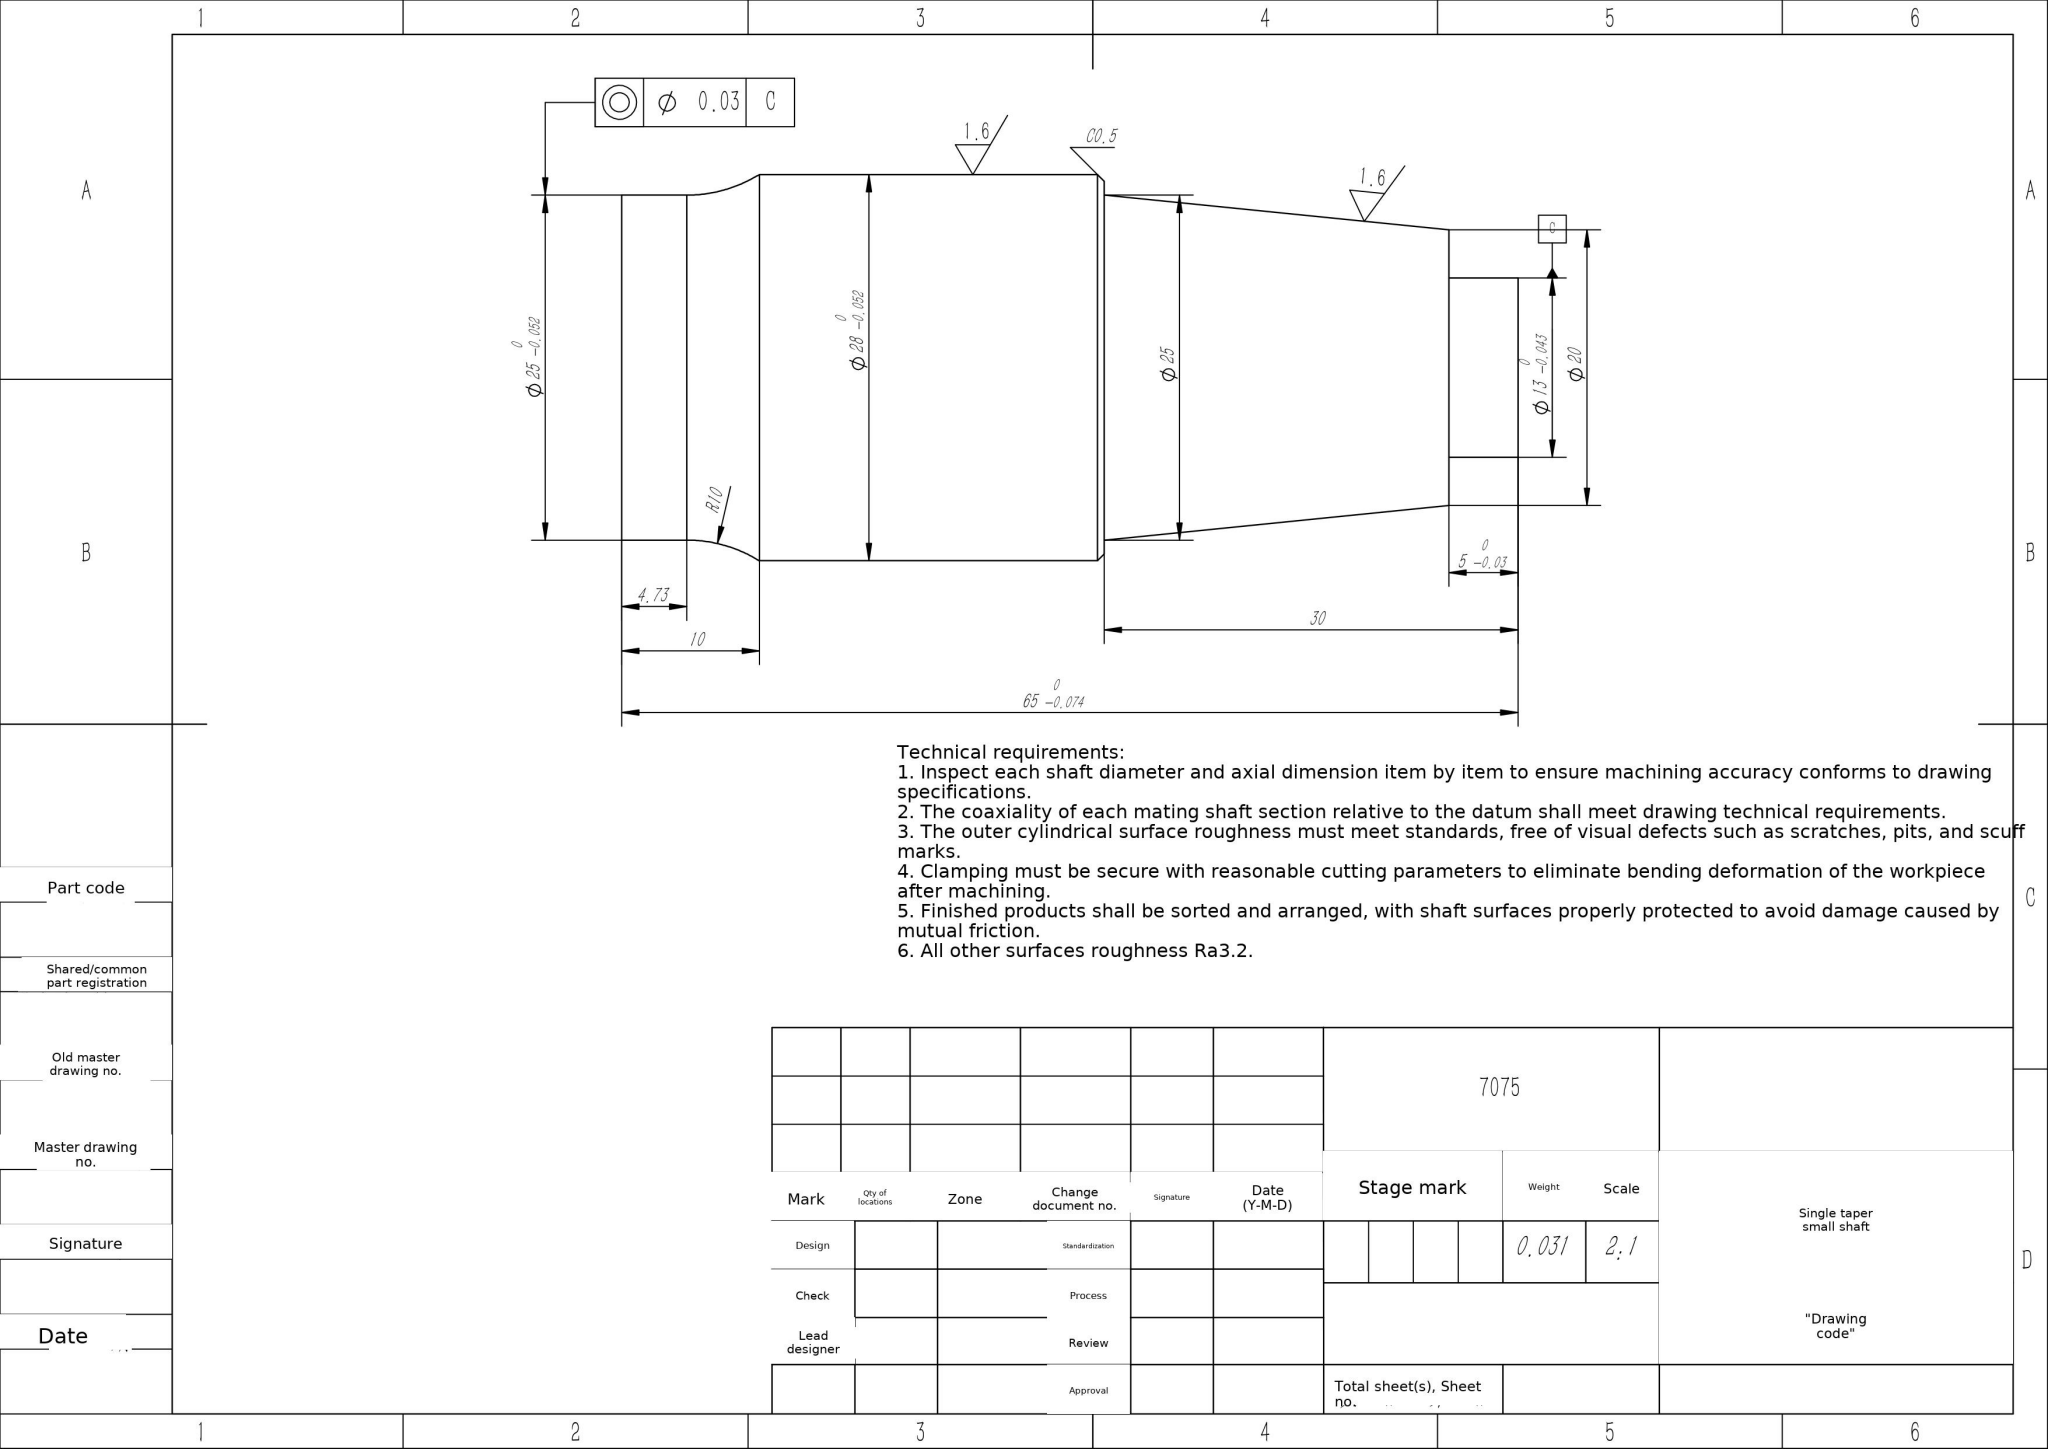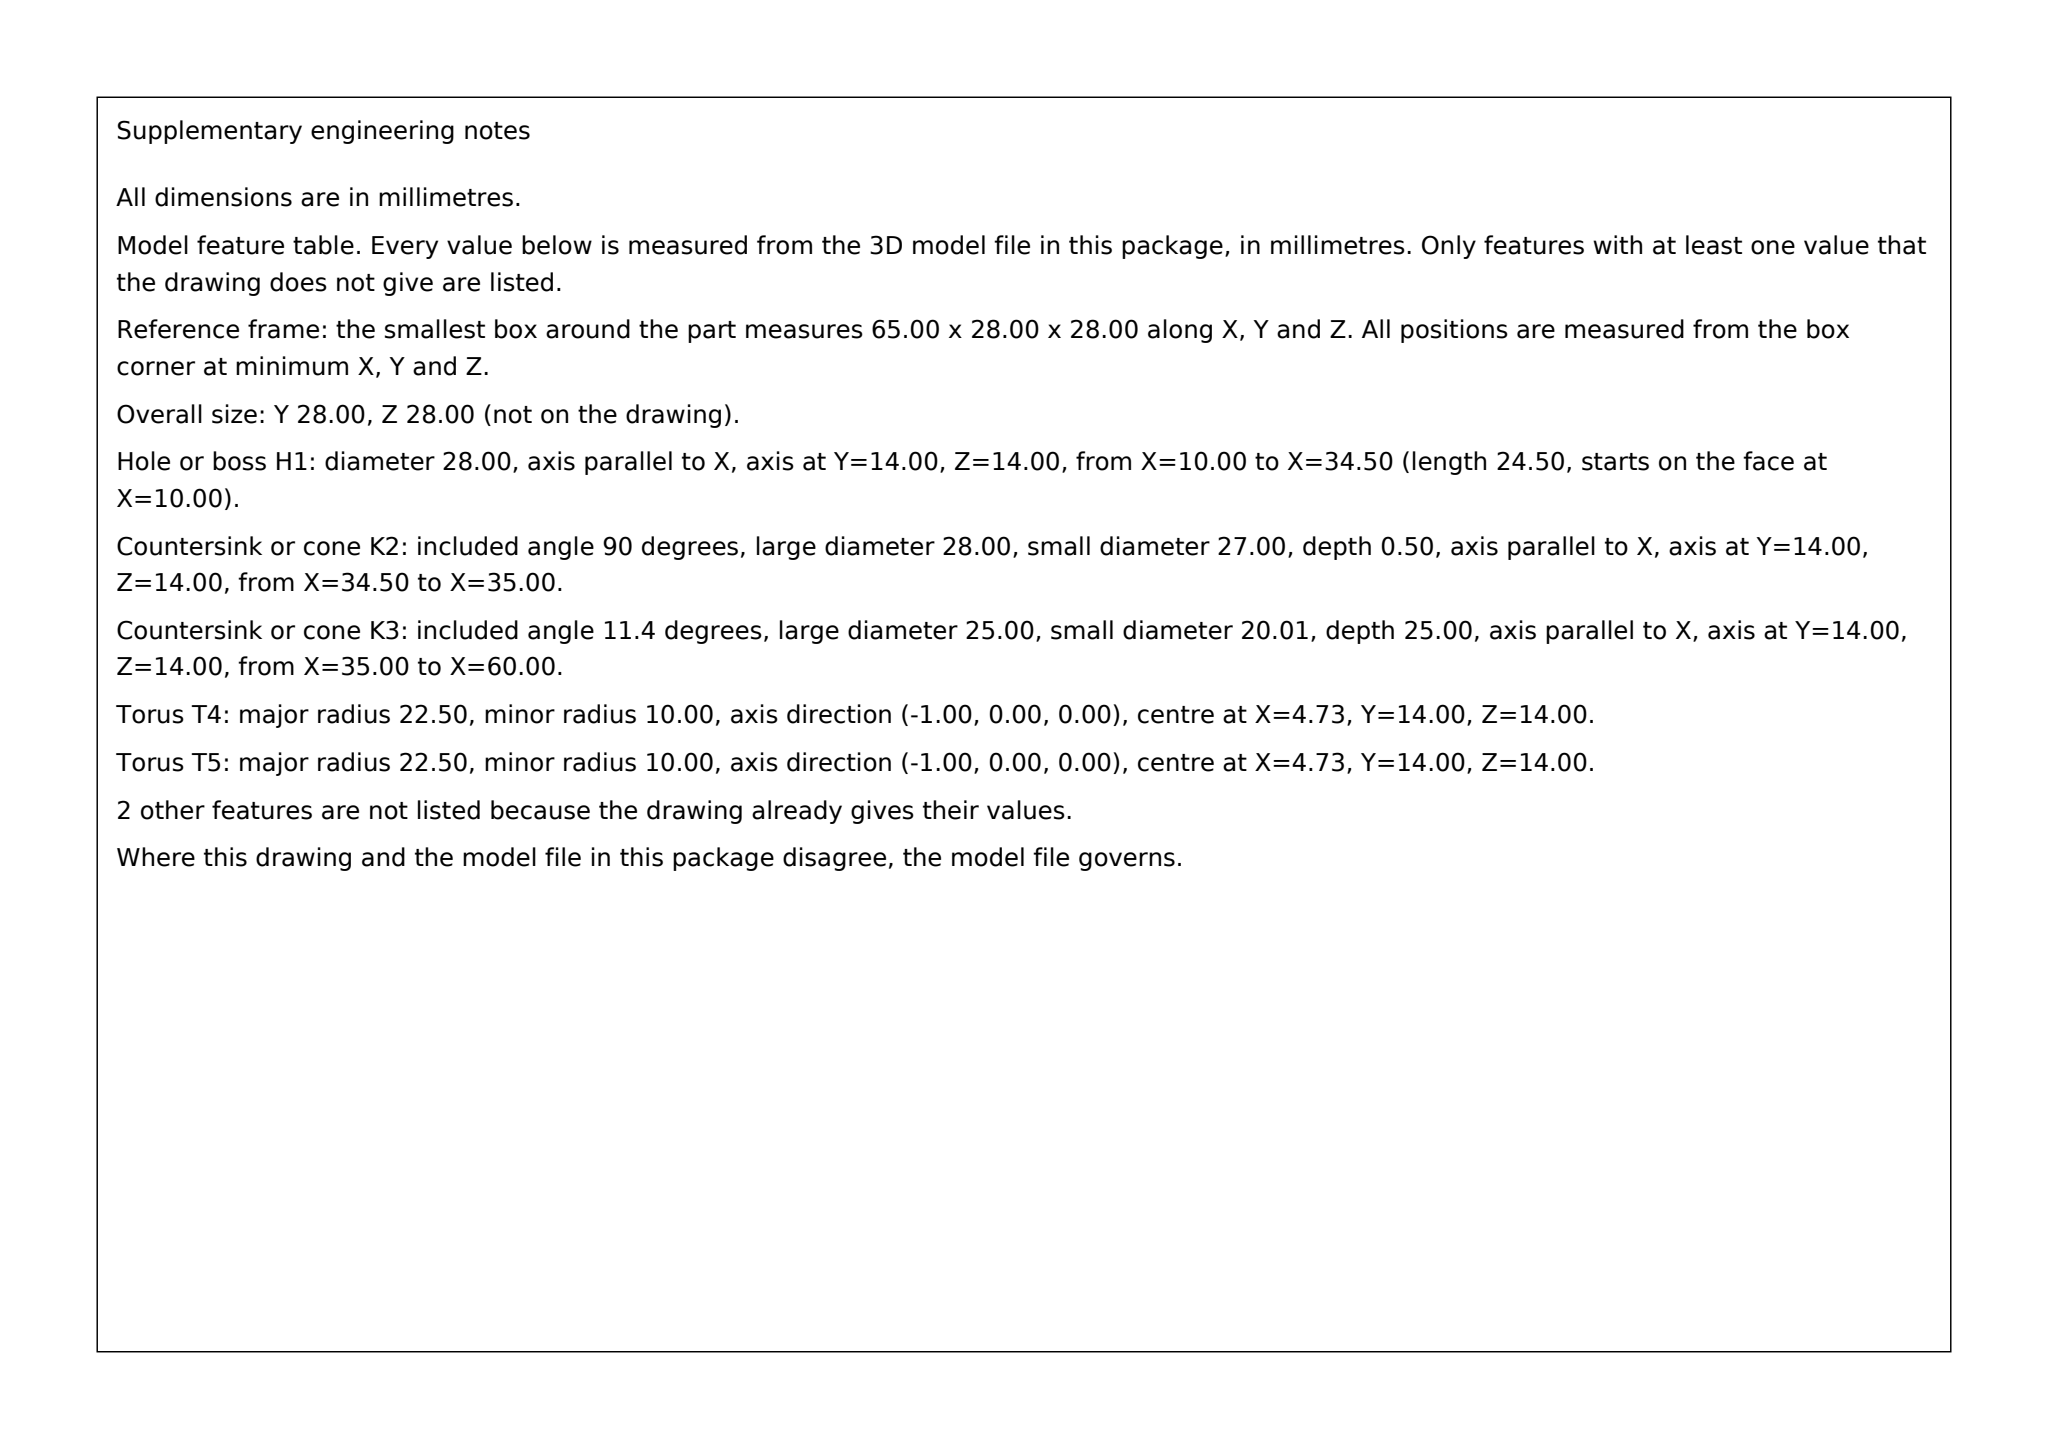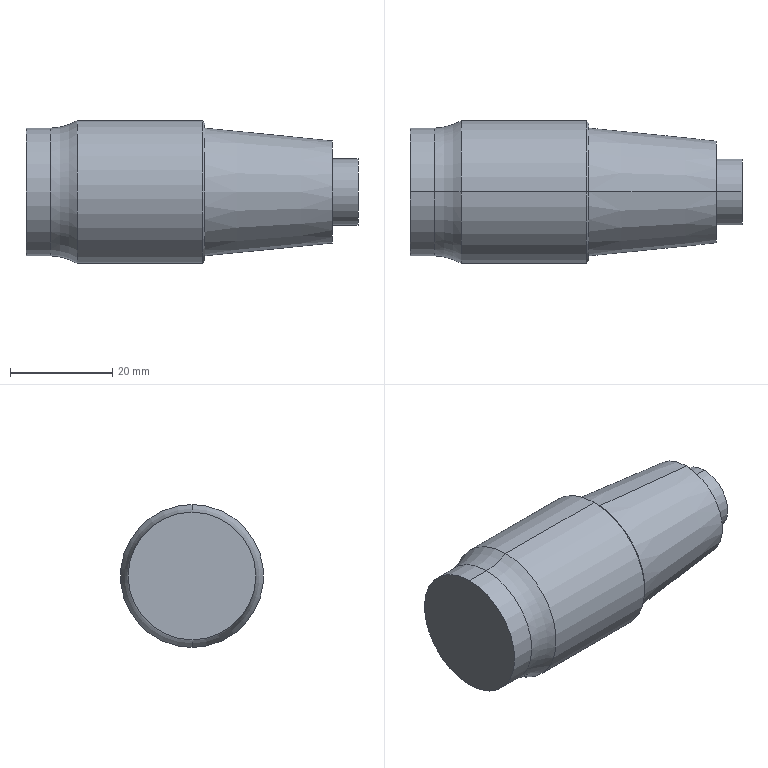Part | SolidWorks | mm | material 7075 | 1 solid | 16 faces | box 65 x 28 x 28 mm | volume 31144 mm3 | cylinder 6 | cone 4 | plane 4 | torus 2 | commonest cylinder face diameters 25 x2 13 x2 28 x2
build123d program:
from build123d import *


with BuildPart() as part:
    # Model → Revolve1 (revolve)
    with BuildSketch(Plane.XY, mode=Mode.PRIVATE) as revolve1_sk:
        with BuildLine():
            Line((-65.059, 12.982), (-65.059, 11.982))
            Line((-65.059, 11.982), (-40.059, 9.482))
            Line((-40.059, 9.482), (-40.059, 5.982))
            Line((-40.059, 5.982), (-35.059, 5.982))
            Line((-35.059, 5.982), (-35.059, -0.5183))
            Line((-35.059, -0.5183), (-100.059, -0.5183))
            Line((-100.059, -0.5183), (-100.059, 11.982))
            Line((-100.059, 11.982), (-95.327, 11.982))
            ThreePointArc((-95.327, 11.982), (-92.588, 12.364), (-90.059, 13.482))
            Line((-90.059, 13.482), (-65.559, 13.482))
            Line((-65.559, 13.482), (-65.059, 12.982))
        make_face()
    revolve(revolve1_sk.sketch.rotate(Axis((-100.059, -0.5183, 0), (1, 0, 0)), 90), axis=Axis((-100.059, -0.5183, 0), (1, 0, 0)))


solid = part.part
STEP:
#1=CARTESIAN_POINT('',(-95.327,-0.5183,12.5));
#2=VERTEX_POINT('',#1);
#3=CARTESIAN_POINT('',(-95.327,-0.5183,-12.5));
#4=VERTEX_POINT('',#3);
#5=CARTESIAN_POINT('',(-95.327,-0.5183,0.));
#6=DIRECTION('',(-1.,0.,0.));
#7=DIRECTION('',(0.,0.,1.));
#8=AXIS2_PLACEMENT_3D('',#5,#6,#7);
#9=CIRCLE('',#8,12.5);
#10=EDGE_CURVE('',#2,#4,#9,.T.);
#11=ORIENTED_EDGE('',*,*,#10,.T.);
#12=CARTESIAN_POINT('',(-100.059,-0.5183,-12.5));
#13=VERTEX_POINT('',#12);
#14=CARTESIAN_POINT('',(-100.059,-0.5183,-12.5));
#15=DIRECTION('',(-1.,0.,0.));
#16=VECTOR('',#15,1000.);
#17=LINE('',#14,#16);
#18=EDGE_CURVE('',#4,#13,#17,.T.);
#19=ORIENTED_EDGE('',*,*,#18,.T.);
#20=CARTESIAN_POINT('',(-100.059,-0.5183,12.5));
#21=VERTEX_POINT('',#20);
#22=CARTESIAN_POINT('',(-100.059,-0.5183,0.));
#23=DIRECTION('',(-1.,0.,0.));
#24=DIRECTION('',(0.,0.,1.));
#25=AXIS2_PLACEMENT_3D('',#22,#23,#24);
#26=CIRCLE('',#25,12.5);
#27=EDGE_CURVE('',#21,#13,#26,.T.);
#28=ORIENTED_EDGE('',*,*,#27,.F.);
#29=CARTESIAN_POINT('',(-100.059,-0.5183,12.5));
#30=DIRECTION('',(-1.,0.,0.));
#31=VECTOR('',#30,1000.);
#32=LINE('',#29,#31);
#33=EDGE_CURVE('',#2,#21,#32,.T.);
#34=ORIENTED_EDGE('',*,*,#33,.F.);
#35=EDGE_LOOP('',(#11,#19,#28,#34));
#36=FACE_OUTER_BOUND('',#35,.T.);
#37=CARTESIAN_POINT('',(-100.059,-0.5183,0.));
#38=DIRECTION('',(-1.,0.,0.));
#39=DIRECTION('',(0.,0.,1.));
#40=AXIS2_PLACEMENT_3D('',#37,#38,#39);
#41=CYLINDRICAL_SURFACE('',#40,12.5);
#42=ADVANCED_FACE('',(#36),#41,.T.);
#43=CARTESIAN_POINT('',(-35.059,-0.5183,6.5));
#44=VERTEX_POINT('',#43);
#45=CARTESIAN_POINT('',(-35.059,-0.5183,-6.5));
#46=VERTEX_POINT('',#45);
#47=CARTESIAN_POINT('',(-35.059,-0.5183,0.));
#48=DIRECTION('',(-1.,0.,0.));
#49=DIRECTION('',(0.,0.,1.));
#50=AXIS2_PLACEMENT_3D('',#47,#48,#49);
#51=CIRCLE('',#50,6.5);
#52=EDGE_CURVE('',#44,#46,#51,.T.);
#53=ORIENTED_EDGE('',*,*,#52,.T.);
#54=CARTESIAN_POINT('',(-40.059,-0.5183,-6.5));
#55=VERTEX_POINT('',#54);
#56=CARTESIAN_POINT('',(-100.059,-0.5183,-6.5));
#57=DIRECTION('',(-1.,0.,0.));
#58=VECTOR('',#57,1000.);
#59=LINE('',#56,#58);
#60=EDGE_CURVE('',#46,#55,#59,.T.);
#61=ORIENTED_EDGE('',*,*,#60,.T.);
#62=CARTESIAN_POINT('',(-40.059,-0.5183,6.5));
#63=VERTEX_POINT('',#62);
#64=CARTESIAN_POINT('',(-40.059,-0.5183,0.));
#65=DIRECTION('',(-1.,0.,0.));
#66=DIRECTION('',(0.,0.,1.));
#67=AXIS2_PLACEMENT_3D('',#64,#65,#66);
#68=CIRCLE('',#67,6.5);
#69=EDGE_CURVE('',#63,#55,#68,.T.);
#70=ORIENTED_EDGE('',*,*,#69,.F.);
#71=CARTESIAN_POINT('',(-100.059,-0.5183,6.5));
#72=DIRECTION('',(-1.,0.,0.));
#73=VECTOR('',#72,1000.);
#74=LINE('',#71,#73);
#75=EDGE_CURVE('',#44,#63,#74,.T.);
#76=ORIENTED_EDGE('',*,*,#75,.F.);
#77=EDGE_LOOP('',(#53,#61,#70,#76));
#78=FACE_OUTER_BOUND('',#77,.T.);
#79=CARTESIAN_POINT('',(-100.059,-0.5183,0.));
#80=DIRECTION('',(-1.,0.,0.));
#81=DIRECTION('',(0.,0.,1.));
#82=AXIS2_PLACEMENT_3D('',#79,#80,#81);
#83=CYLINDRICAL_SURFACE('',#82,6.5);
#84=ADVANCED_FACE('',(#78),#83,.T.);
#85=CARTESIAN_POINT('',(-40.059,-0.5183,10.));
#86=VERTEX_POINT('',#85);
#87=CARTESIAN_POINT('',(-40.059,-0.5183,-10.));
#88=VERTEX_POINT('',#87);
#89=CARTESIAN_POINT('',(-40.059,-0.5183,0.));
#90=DIRECTION('',(-1.,0.,0.));
#91=DIRECTION('',(0.,0.,1.));
#92=AXIS2_PLACEMENT_3D('',#89,#90,#91);
#93=CIRCLE('',#92,10.);
#94=EDGE_CURVE('',#86,#88,#93,.T.);
#95=ORIENTED_EDGE('',*,*,#94,.T.);
#96=CARTESIAN_POINT('',(-65.059,-0.5183,-12.5));
#97=VERTEX_POINT('',#96);
#98=CARTESIAN_POINT('',(-40.059,-0.5183,-10.));
#99=DIRECTION('',(-0.995,0.,-0.0995));
#100=VECTOR('',#99,1000.);
#101=LINE('',#98,#100);
#102=EDGE_CURVE('',#88,#97,#101,.T.);
#103=ORIENTED_EDGE('',*,*,#102,.T.);
#104=CARTESIAN_POINT('',(-65.059,-0.5183,12.5));
#105=VERTEX_POINT('',#104);
#106=CARTESIAN_POINT('',(-65.059,-0.5183,0.));
#107=DIRECTION('',(-1.,0.,0.));
#108=DIRECTION('',(0.,0.,1.));
#109=AXIS2_PLACEMENT_3D('',#106,#107,#108);
#110=CIRCLE('',#109,12.5);
#111=EDGE_CURVE('',#105,#97,#110,.T.);
#112=ORIENTED_EDGE('',*,*,#111,.F.);
#113=CARTESIAN_POINT('',(-40.059,-0.5183,10.));
#114=DIRECTION('',(-0.995,0.,0.0995));
#115=VECTOR('',#114,1000.);
#116=LINE('',#113,#115);
#117=EDGE_CURVE('',#86,#105,#116,.T.);
#118=ORIENTED_EDGE('',*,*,#117,.F.);
#119=EDGE_LOOP('',(#95,#103,#112,#118));
#120=FACE_OUTER_BOUND('',#119,.T.);
#121=CARTESIAN_POINT('',(-40.059,-0.5183,0.));
#122=DIRECTION('',(-1.,0.,0.));
#123=DIRECTION('',(0.,0.,1.));
#124=AXIS2_PLACEMENT_3D('',#121,#122,#123);
#125=CONICAL_SURFACE('',#124,10.,0.09967);
#126=ADVANCED_FACE('',(#120),#125,.T.);
#127=CARTESIAN_POINT('',(-65.059,-0.5183,13.5));
#128=VERTEX_POINT('',#127);
#129=CARTESIAN_POINT('',(-65.059,-0.5183,-13.5));
#130=VERTEX_POINT('',#129);
#131=CARTESIAN_POINT('',(-65.059,-0.5183,0.));
#132=DIRECTION('',(-1.,0.,0.));
#133=DIRECTION('',(0.,0.,1.));
#134=AXIS2_PLACEMENT_3D('',#131,#132,#133);
#135=CIRCLE('',#134,13.5);
#136=EDGE_CURVE('',#128,#130,#135,.T.);
#137=ORIENTED_EDGE('',*,*,#136,.T.);
#138=CARTESIAN_POINT('',(-65.559,-0.5183,-14.));
#139=VERTEX_POINT('',#138);
#140=CARTESIAN_POINT('',(-65.059,-0.5183,-13.5));
#141=DIRECTION('',(-0.7071,0.,-0.7071));
#142=VECTOR('',#141,1000.);
#143=LINE('',#140,#142);
#144=EDGE_CURVE('',#130,#139,#143,.T.);
#145=ORIENTED_EDGE('',*,*,#144,.T.);
#146=CARTESIAN_POINT('',(-65.559,-0.5183,14.));
#147=VERTEX_POINT('',#146);
#148=CARTESIAN_POINT('',(-65.559,-0.5183,0.));
#149=DIRECTION('',(-1.,0.,0.));
#150=DIRECTION('',(0.,0.,1.));
#151=AXIS2_PLACEMENT_3D('',#148,#149,#150);
#152=CIRCLE('',#151,14.);
#153=EDGE_CURVE('',#147,#139,#152,.T.);
#154=ORIENTED_EDGE('',*,*,#153,.F.);
#155=CARTESIAN_POINT('',(-65.059,-0.5183,13.5));
#156=DIRECTION('',(-0.7071,0.,0.7071));
#157=VECTOR('',#156,1000.);
#158=LINE('',#155,#157);
#159=EDGE_CURVE('',#128,#147,#158,.T.);
#160=ORIENTED_EDGE('',*,*,#159,.F.);
#161=EDGE_LOOP('',(#137,#145,#154,#160));
#162=FACE_OUTER_BOUND('',#161,.T.);
#163=CARTESIAN_POINT('',(-65.059,-0.5183,0.));
#164=DIRECTION('',(-1.,0.,0.));
#165=DIRECTION('',(0.,0.,1.));
#166=AXIS2_PLACEMENT_3D('',#163,#164,#165);
#167=CONICAL_SURFACE('',#166,13.5,0.7854);
#168=ADVANCED_FACE('',(#162),#167,.T.);
#169=ORIENTED_EDGE('',*,*,#153,.T.);
#170=CARTESIAN_POINT('',(-90.059,-0.5183,-14.));
#171=VERTEX_POINT('',#170);
#172=CARTESIAN_POINT('',(-100.059,-0.5183,-14.));
#173=DIRECTION('',(-1.,0.,0.));
#174=VECTOR('',#173,1000.);
#175=LINE('',#172,#174);
#176=EDGE_CURVE('',#139,#171,#175,.T.);
#177=ORIENTED_EDGE('',*,*,#176,.T.);
#178=CARTESIAN_POINT('',(-90.059,-0.5183,14.));
#179=VERTEX_POINT('',#178);
#180=CARTESIAN_POINT('',(-90.059,-0.5183,0.));
#181=DIRECTION('',(-1.,0.,0.));
#182=DIRECTION('',(0.,0.,1.));
#183=AXIS2_PLACEMENT_3D('',#180,#181,#182);
#184=CIRCLE('',#183,14.);
#185=EDGE_CURVE('',#179,#171,#184,.T.);
#186=ORIENTED_EDGE('',*,*,#185,.F.);
#187=CARTESIAN_POINT('',(-100.059,-0.5183,14.));
#188=DIRECTION('',(-1.,0.,0.));
#189=VECTOR('',#188,1000.);
#190=LINE('',#187,#189);
#191=EDGE_CURVE('',#147,#179,#190,.T.);
#192=ORIENTED_EDGE('',*,*,#191,.F.);
#193=EDGE_LOOP('',(#169,#177,#186,#192));
#194=FACE_OUTER_BOUND('',#193,.T.);
#195=CARTESIAN_POINT('',(-100.059,-0.5183,0.));
#196=DIRECTION('',(-1.,0.,0.));
#197=DIRECTION('',(0.,0.,1.));
#198=AXIS2_PLACEMENT_3D('',#195,#196,#197);
#199=CYLINDRICAL_SURFACE('',#198,14.);
#200=ADVANCED_FACE('',(#194),#199,.T.);
#201=CARTESIAN_POINT('',(-95.327,-0.5183,0.));
#202=DIRECTION('',(-1.,0.,0.));
#203=DIRECTION('',(0.,0.,1.));
#204=AXIS2_PLACEMENT_3D('',#201,#202,#203);
#205=CIRCLE('',#204,12.5);
#206=EDGE_CURVE('',#4,#2,#205,.T.);
#207=ORIENTED_EDGE('',*,*,#206,.F.);
#208=CARTESIAN_POINT('',(-95.327,-0.5183,-22.5));
#209=DIRECTION('',(0.,1.,0.));
#210=DIRECTION('',(0.,-0.,1.));
#211=AXIS2_PLACEMENT_3D('',#208,#209,#210);
#212=CIRCLE('',#211,10.);
#213=EDGE_CURVE('',#4,#171,#212,.T.);
#214=ORIENTED_EDGE('',*,*,#213,.T.);
#215=CARTESIAN_POINT('',(-90.059,-0.5183,0.));
#216=DIRECTION('',(-1.,0.,0.));
#217=DIRECTION('',(0.,0.,1.));
#218=AXIS2_PLACEMENT_3D('',#215,#216,#217);
#219=CIRCLE('',#218,14.);
#220=EDGE_CURVE('',#171,#179,#219,.T.);
#221=ORIENTED_EDGE('',*,*,#220,.T.);
#222=CARTESIAN_POINT('',(-95.327,-0.5183,22.5));
#223=DIRECTION('',(0.,-1.,0.));
#224=DIRECTION('',(0.,0.,-1.));
#225=AXIS2_PLACEMENT_3D('',#222,#223,#224);
#226=CIRCLE('',#225,10.);
#227=EDGE_CURVE('',#2,#179,#226,.T.);
#228=ORIENTED_EDGE('',*,*,#227,.F.);
#229=EDGE_LOOP('',(#207,#214,#221,#228));
#230=FACE_OUTER_BOUND('',#229,.T.);
#231=CARTESIAN_POINT('',(-95.327,-0.5183,0.));
#232=DIRECTION('',(-1.,0.,0.));
#233=DIRECTION('',(0.,0.,1.));
#234=AXIS2_PLACEMENT_3D('',#231,#232,#233);
#235=TOROIDAL_SURFACE('',#234,22.5,10.);
#236=ADVANCED_FACE('',(#230),#235,.F.);
#237=ORIENTED_EDGE('',*,*,#213,.F.);
#238=ORIENTED_EDGE('',*,*,#10,.F.);
#239=ORIENTED_EDGE('',*,*,#227,.T.);
#240=ORIENTED_EDGE('',*,*,#185,.T.);
#241=EDGE_LOOP('',(#237,#238,#239,#240));
#242=FACE_OUTER_BOUND('',#241,.T.);
#243=CARTESIAN_POINT('',(-95.327,-0.5183,0.));
#244=DIRECTION('',(-1.,0.,0.));
#245=DIRECTION('',(0.,0.,1.));
#246=AXIS2_PLACEMENT_3D('',#243,#244,#245);
#247=TOROIDAL_SURFACE('',#246,22.5,10.);
#248=ADVANCED_FACE('',(#242),#247,.F.);
#249=ORIENTED_EDGE('',*,*,#176,.F.);
#250=CARTESIAN_POINT('',(-65.559,-0.5183,0.));
#251=DIRECTION('',(-1.,0.,0.));
#252=DIRECTION('',(0.,0.,1.));
#253=AXIS2_PLACEMENT_3D('',#250,#251,#252);
#254=CIRCLE('',#253,14.);
#255=EDGE_CURVE('',#139,#147,#254,.T.);
#256=ORIENTED_EDGE('',*,*,#255,.T.);
#257=ORIENTED_EDGE('',*,*,#191,.T.);
#258=ORIENTED_EDGE('',*,*,#220,.F.);
#259=EDGE_LOOP('',(#249,#256,#257,#258));
#260=FACE_OUTER_BOUND('',#259,.T.);
#261=CARTESIAN_POINT('',(-100.059,-0.5183,0.));
#262=DIRECTION('',(-1.,0.,0.));
#263=DIRECTION('',(0.,0.,1.));
#264=AXIS2_PLACEMENT_3D('',#261,#262,#263);
#265=CYLINDRICAL_SURFACE('',#264,14.);
#266=ADVANCED_FACE('',(#260),#265,.T.);
#267=ORIENTED_EDGE('',*,*,#144,.F.);
#268=CARTESIAN_POINT('',(-65.059,-0.5183,0.));
#269=DIRECTION('',(-1.,0.,0.));
#270=DIRECTION('',(0.,0.,1.));
#271=AXIS2_PLACEMENT_3D('',#268,#269,#270);
#272=CIRCLE('',#271,13.5);
#273=EDGE_CURVE('',#130,#128,#272,.T.);
#274=ORIENTED_EDGE('',*,*,#273,.T.);
#275=ORIENTED_EDGE('',*,*,#159,.T.);
#276=ORIENTED_EDGE('',*,*,#255,.F.);
#277=EDGE_LOOP('',(#267,#274,#275,#276));
#278=FACE_OUTER_BOUND('',#277,.T.);
#279=CARTESIAN_POINT('',(-65.059,-0.5183,0.));
#280=DIRECTION('',(-1.,0.,0.));
#281=DIRECTION('',(0.,0.,1.));
#282=AXIS2_PLACEMENT_3D('',#279,#280,#281);
#283=CONICAL_SURFACE('',#282,13.5,0.7854);
#284=ADVANCED_FACE('',(#278),#283,.T.);
#285=ORIENTED_EDGE('',*,*,#136,.F.);
#286=ORIENTED_EDGE('',*,*,#273,.F.);
#287=EDGE_LOOP('',(#285,#286));
#288=FACE_OUTER_BOUND('',#287,.T.);
#289=ORIENTED_EDGE('',*,*,#111,.T.);
#290=CARTESIAN_POINT('',(-65.059,-0.5183,0.));
#291=DIRECTION('',(-1.,0.,0.));
#292=DIRECTION('',(0.,0.,1.));
#293=AXIS2_PLACEMENT_3D('',#290,#291,#292);
#294=CIRCLE('',#293,12.5);
#295=EDGE_CURVE('',#97,#105,#294,.T.);
#296=ORIENTED_EDGE('',*,*,#295,.T.);
#297=EDGE_LOOP('',(#289,#296));
#298=FACE_BOUND('',#297,.T.);
#299=CARTESIAN_POINT('',(-65.059,12.982,0.));
#300=DIRECTION('',(-1.,0.,0.));
#301=DIRECTION('',(0.,0.,1.));
#302=AXIS2_PLACEMENT_3D('',#299,#300,#301);
#303=PLANE('',#302);
#304=ADVANCED_FACE('',(#288,#298),#303,.F.);
#305=ORIENTED_EDGE('',*,*,#102,.F.);
#306=CARTESIAN_POINT('',(-40.059,-0.5183,0.));
#307=DIRECTION('',(-1.,0.,0.));
#308=DIRECTION('',(0.,0.,1.));
#309=AXIS2_PLACEMENT_3D('',#306,#307,#308);
#310=CIRCLE('',#309,10.);
#311=EDGE_CURVE('',#88,#86,#310,.T.);
#312=ORIENTED_EDGE('',*,*,#311,.T.);
#313=ORIENTED_EDGE('',*,*,#117,.T.);
#314=ORIENTED_EDGE('',*,*,#295,.F.);
#315=EDGE_LOOP('',(#305,#312,#313,#314));
#316=FACE_OUTER_BOUND('',#315,.T.);
#317=CARTESIAN_POINT('',(-40.059,-0.5183,0.));
#318=DIRECTION('',(-1.,0.,0.));
#319=DIRECTION('',(0.,0.,1.));
#320=AXIS2_PLACEMENT_3D('',#317,#318,#319);
#321=CONICAL_SURFACE('',#320,10.,0.09967);
#322=ADVANCED_FACE('',(#316),#321,.T.);
#323=ORIENTED_EDGE('',*,*,#94,.F.);
#324=ORIENTED_EDGE('',*,*,#311,.F.);
#325=EDGE_LOOP('',(#323,#324));
#326=FACE_OUTER_BOUND('',#325,.T.);
#327=ORIENTED_EDGE('',*,*,#69,.T.);
#328=CARTESIAN_POINT('',(-40.059,-0.5183,0.));
#329=DIRECTION('',(-1.,0.,0.));
#330=DIRECTION('',(0.,0.,1.));
#331=AXIS2_PLACEMENT_3D('',#328,#329,#330);
#332=CIRCLE('',#331,6.5);
#333=EDGE_CURVE('',#55,#63,#332,.T.);
#334=ORIENTED_EDGE('',*,*,#333,.T.);
#335=EDGE_LOOP('',(#327,#334));
#336=FACE_BOUND('',#335,.T.);
#337=CARTESIAN_POINT('',(-40.059,9.482,0.));
#338=DIRECTION('',(-1.,0.,0.));
#339=DIRECTION('',(0.,0.,1.));
#340=AXIS2_PLACEMENT_3D('',#337,#338,#339);
#341=PLANE('',#340);
#342=ADVANCED_FACE('',(#326,#336),#341,.F.);
#343=ORIENTED_EDGE('',*,*,#60,.F.);
#344=CARTESIAN_POINT('',(-35.059,-0.5183,0.));
#345=DIRECTION('',(-1.,0.,0.));
#346=DIRECTION('',(0.,0.,1.));
#347=AXIS2_PLACEMENT_3D('',#344,#345,#346);
#348=CIRCLE('',#347,6.5);
#349=EDGE_CURVE('',#46,#44,#348,.T.);
#350=ORIENTED_EDGE('',*,*,#349,.T.);
#351=ORIENTED_EDGE('',*,*,#75,.T.);
#352=ORIENTED_EDGE('',*,*,#333,.F.);
#353=EDGE_LOOP('',(#343,#350,#351,#352));
#354=FACE_OUTER_BOUND('',#353,.T.);
#355=CARTESIAN_POINT('',(-100.059,-0.5183,0.));
#356=DIRECTION('',(-1.,0.,0.));
#357=DIRECTION('',(0.,0.,1.));
#358=AXIS2_PLACEMENT_3D('',#355,#356,#357);
#359=CYLINDRICAL_SURFACE('',#358,6.5);
#360=ADVANCED_FACE('',(#354),#359,.T.);
#361=ORIENTED_EDGE('',*,*,#52,.F.);
#362=ORIENTED_EDGE('',*,*,#349,.F.);
#363=EDGE_LOOP('',(#361,#362));
#364=FACE_OUTER_BOUND('',#363,.T.);
#365=CARTESIAN_POINT('',(-35.059,5.982,0.));
#366=DIRECTION('',(-1.,0.,0.));
#367=DIRECTION('',(0.,0.,1.));
#368=AXIS2_PLACEMENT_3D('',#365,#366,#367);
#369=PLANE('',#368);
#370=ADVANCED_FACE('',(#364),#369,.F.);
#371=ORIENTED_EDGE('',*,*,#27,.T.);
#372=CARTESIAN_POINT('',(-100.059,-0.5183,0.));
#373=DIRECTION('',(-1.,0.,0.));
#374=DIRECTION('',(0.,0.,1.));
#375=AXIS2_PLACEMENT_3D('',#372,#373,#374);
#376=CIRCLE('',#375,12.5);
#377=EDGE_CURVE('',#13,#21,#376,.T.);
#378=ORIENTED_EDGE('',*,*,#377,.T.);
#379=EDGE_LOOP('',(#371,#378));
#380=FACE_OUTER_BOUND('',#379,.T.);
#381=CARTESIAN_POINT('',(-100.059,11.982,0.));
#382=DIRECTION('',(1.,0.,0.));
#383=DIRECTION('',(0.,0.,-1.));
#384=AXIS2_PLACEMENT_3D('',#381,#382,#383);
#385=PLANE('',#384);
#386=ADVANCED_FACE('',(#380),#385,.F.);
#387=ORIENTED_EDGE('',*,*,#18,.F.);
#388=ORIENTED_EDGE('',*,*,#206,.T.);
#389=ORIENTED_EDGE('',*,*,#33,.T.);
#390=ORIENTED_EDGE('',*,*,#377,.F.);
#391=EDGE_LOOP('',(#387,#388,#389,#390));
#392=FACE_OUTER_BOUND('',#391,.T.);
#393=CARTESIAN_POINT('',(-100.059,-0.5183,0.));
#394=DIRECTION('',(-1.,0.,0.));
#395=DIRECTION('',(0.,0.,1.));
#396=AXIS2_PLACEMENT_3D('',#393,#394,#395);
#397=CYLINDRICAL_SURFACE('',#396,12.5);
#398=ADVANCED_FACE('',(#392),#397,.T.);
#399=CLOSED_SHELL('',(#42,#84,#126,#168,#200,#236,#248,#266,#284,#304,#322,#342,#360,#370,#386,#398));
#400=MANIFOLD_SOLID_BREP('',#399);
#401=CARTESIAN_POINT('',(0.,0.,0.));
#402=DIRECTION('',(0.,0.,1.));
#403=DIRECTION('',(1.,0.,0.));
#404=AXIS2_PLACEMENT_3D('',#401,#402,#403);
#405=(LENGTH_UNIT()NAMED_UNIT(*)SI_UNIT(.MILLI.,.METRE.));
#406=UNCERTAINTY_MEASURE_WITH_UNIT(LENGTH_MEASURE(0.00001),#405,'','');
#407=(NAMED_UNIT(*)PLANE_ANGLE_UNIT()SI_UNIT($,.RADIAN.));
#408=(NAMED_UNIT(*)SI_UNIT($,.STERADIAN.)SOLID_ANGLE_UNIT());
#409=(GEOMETRIC_REPRESENTATION_CONTEXT(3)GLOBAL_UNCERTAINTY_ASSIGNED_CONTEXT((#406))GLOBAL_UNIT_ASSIGNED_CONTEXT((#405,#407,#408))REPRESENTATION_CONTEXT('',''));
#410=ADVANCED_BREP_SHAPE_REPRESENTATION('',(#400,#404),#409);